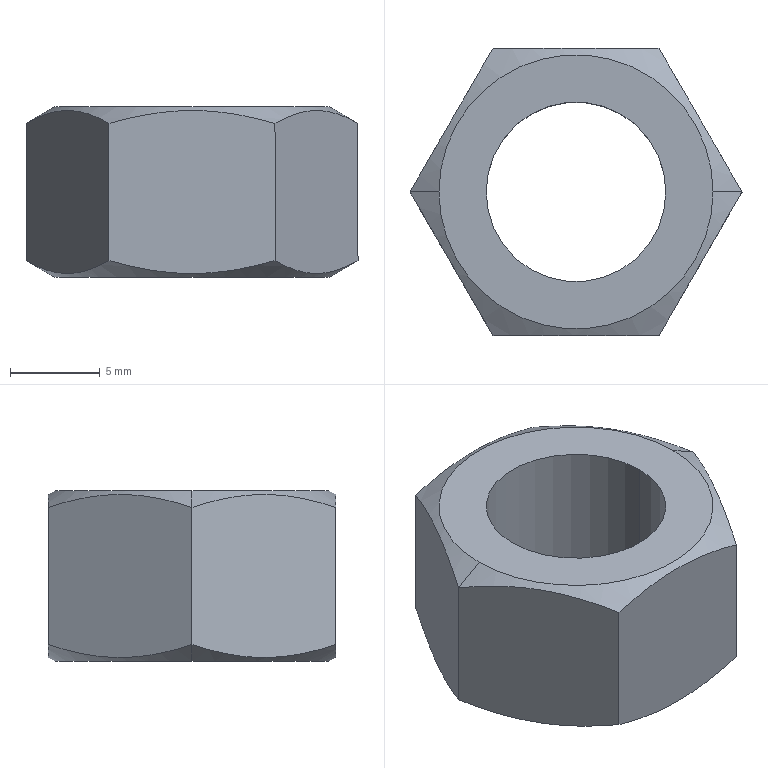Component | SolidWorks | hexagon nuts grade c gb-1 | 1 solid | 14 faces | box 18.48 x 16 x 9.5 mm | volume 1338 mm3 | plane 8 | cone 4 | cylinder 2 | commonest cylinder face diameters 10 x2
STEP:
#1=COLOUR_RGB('',0.7922,0.8196,0.9333);
#2=FILL_AREA_STYLE_COLOUR('',#1);
#3=FILL_AREA_STYLE('',(#2));
#4=SURFACE_STYLE_FILL_AREA(#3);
#5=SURFACE_SIDE_STYLE('',(#4));
#6=SURFACE_STYLE_USAGE(.BOTH.,#5);
#7=PRESENTATION_STYLE_ASSIGNMENT((#6));
#8=CARTESIAN_POINT('',(2.439,-3.29,-4.35));
#9=VERTEX_POINT('',#8);
#10=CARTESIAN_POINT('',(3.039,-3.29,-4.35));
#11=VERTEX_POINT('',#10);
#12=CARTESIAN_POINT('',(2.739,-3.29,-4.35));
#13=DIRECTION('',(0.,0.,-1.));
#14=DIRECTION('',(-1.,0.,0.));
#15=AXIS2_PLACEMENT_3D('',#12,#13,#14);
#16=CIRCLE('',#15,0.3002);
#17=EDGE_CURVE('',#9,#11,#16,.T.);
#18=ORIENTED_EDGE('',*,*,#17,.T.);
#19=CARTESIAN_POINT('',(3.103,-3.29,-4.387));
#20=VERTEX_POINT('',#19);
#21=CARTESIAN_POINT('',(3.039,-3.29,-4.35));
#22=DIRECTION('',(0.866,0.,-0.5));
#23=VECTOR('',#22,39.37);
#24=LINE('',#21,#23);
#25=EDGE_CURVE('',#11,#20,#24,.T.);
#26=ORIENTED_EDGE('',*,*,#25,.T.);
#27=CARTESIAN_POINT('',(2.921,-2.975,-4.387));
#28=VERTEX_POINT('',#27);
#29=CARTESIAN_POINT('',(3.103,-3.29,-4.387));
#30=CARTESIAN_POINT('',(3.088,-3.264,-4.378));
#31=CARTESIAN_POINT('',(3.073,-3.238,-4.371));
#32=CARTESIAN_POINT('',(3.043,-3.186,-4.362));
#33=CARTESIAN_POINT('',(3.027,-3.159,-4.359));
#34=CARTESIAN_POINT('',(3.004,-3.119,-4.359));
#35=CARTESIAN_POINT('',(2.996,-3.106,-4.36));
#36=CARTESIAN_POINT('',(2.981,-3.079,-4.362));
#37=CARTESIAN_POINT('',(2.973,-3.066,-4.364));
#38=CARTESIAN_POINT('',(2.951,-3.027,-4.371));
#39=CARTESIAN_POINT('',(2.936,-3.001,-4.378));
#40=CARTESIAN_POINT('',(2.921,-2.975,-4.387));
#41=B_SPLINE_CURVE_WITH_KNOTS('',3,(#29,#30,#31,#32,#33,#34,#35,#36,#37,#38,#39,#40),.UNSPECIFIED.,.F.,.F.,(4,2,2,2,2,4),(0.00000024,0.002333,0.004665,0.005831,0.006997,0.00933),.UNSPECIFIED.);
#42=EDGE_CURVE('',#20,#28,#41,.T.);
#43=ORIENTED_EDGE('',*,*,#42,.T.);
#44=CARTESIAN_POINT('',(2.557,-2.975,-4.387));
#45=VERTEX_POINT('',#44);
#46=CARTESIAN_POINT('',(2.921,-2.975,-4.387));
#47=CARTESIAN_POINT('',(2.891,-2.975,-4.379));
#48=CARTESIAN_POINT('',(2.862,-2.975,-4.371));
#49=CARTESIAN_POINT('',(2.801,-2.975,-4.362));
#50=CARTESIAN_POINT('',(2.77,-2.975,-4.359));
#51=CARTESIAN_POINT('',(2.708,-2.975,-4.359));
#52=CARTESIAN_POINT('',(2.678,-2.975,-4.362));
#53=CARTESIAN_POINT('',(2.617,-2.975,-4.371));
#54=CARTESIAN_POINT('',(2.587,-2.975,-4.379));
#55=CARTESIAN_POINT('',(2.557,-2.975,-4.387));
#56=B_SPLINE_CURVE_WITH_KNOTS('',3,(#46,#47,#48,#49,#50,#51,#52,#53,#54,#55),.UNSPECIFIED.,.F.,.F.,(4,2,2,2,4),(0.003422,0.005753,0.008084,0.01041,0.01275),.UNSPECIFIED.);
#57=EDGE_CURVE('',#28,#45,#56,.T.);
#58=ORIENTED_EDGE('',*,*,#57,.T.);
#59=CARTESIAN_POINT('',(2.375,-3.29,-4.387));
#60=VERTEX_POINT('',#59);
#61=CARTESIAN_POINT('',(2.557,-2.975,-4.387));
#62=CARTESIAN_POINT('',(2.542,-3.001,-4.378));
#63=CARTESIAN_POINT('',(2.527,-3.026,-4.371));
#64=CARTESIAN_POINT('',(2.497,-3.079,-4.362));
#65=CARTESIAN_POINT('',(2.482,-3.105,-4.359));
#66=CARTESIAN_POINT('',(2.459,-3.145,-4.359));
#67=CARTESIAN_POINT('',(2.451,-3.159,-4.36));
#68=CARTESIAN_POINT('',(2.436,-3.185,-4.362));
#69=CARTESIAN_POINT('',(2.428,-3.199,-4.364));
#70=CARTESIAN_POINT('',(2.405,-3.238,-4.371));
#71=CARTESIAN_POINT('',(2.39,-3.264,-4.378));
#72=CARTESIAN_POINT('',(2.375,-3.29,-4.387));
#73=B_SPLINE_CURVE_WITH_KNOTS('',3,(#61,#62,#63,#64,#65,#66,#67,#68,#69,#70,#71,#72),.UNSPECIFIED.,.F.,.F.,(4,2,2,2,2,4),(0.00000024,0.002333,0.004665,0.005831,0.006997,0.00933),.UNSPECIFIED.);
#74=EDGE_CURVE('',#45,#60,#73,.T.);
#75=ORIENTED_EDGE('',*,*,#74,.T.);
#76=CARTESIAN_POINT('',(2.439,-3.29,-4.35));
#77=DIRECTION('',(-0.866,0.,-0.5));
#78=VECTOR('',#77,39.37);
#79=LINE('',#76,#78);
#80=EDGE_CURVE('',#9,#60,#79,.T.);
#81=ORIENTED_EDGE('',*,*,#80,.F.);
#82=EDGE_LOOP('',(#18,#26,#43,#58,#75,#81));
#83=FACE_OUTER_BOUND('',#82,.T.);
#84=CARTESIAN_POINT('',(2.739,-3.29,-4.35));
#85=DIRECTION('',(0.,0.,-1.));
#86=DIRECTION('',(-1.,0.,0.));
#87=AXIS2_PLACEMENT_3D('',#84,#85,#86);
#88=CONICAL_SURFACE('',#87,0.3002,1.047);
#89=ADVANCED_FACE('',(#83),#88,.T.);
#90=CARTESIAN_POINT('',(2.439,-3.29,-4.724));
#91=VERTEX_POINT('',#90);
#92=CARTESIAN_POINT('',(3.039,-3.29,-4.724));
#93=VERTEX_POINT('',#92);
#94=CARTESIAN_POINT('',(2.739,-3.29,-4.724));
#95=DIRECTION('',(0.,0.,-1.));
#96=DIRECTION('',(-1.,0.,0.));
#97=AXIS2_PLACEMENT_3D('',#94,#95,#96);
#98=CIRCLE('',#97,0.3002);
#99=EDGE_CURVE('',#91,#93,#98,.T.);
#100=ORIENTED_EDGE('',*,*,#99,.F.);
#101=CARTESIAN_POINT('',(2.375,-3.29,-4.688));
#102=VERTEX_POINT('',#101);
#103=CARTESIAN_POINT('',(2.375,-3.29,-4.688));
#104=DIRECTION('',(-0.866,0.,0.5));
#105=VECTOR('',#104,39.37);
#106=LINE('',#103,#105);
#107=EDGE_CURVE('',#91,#102,#106,.T.);
#108=ORIENTED_EDGE('',*,*,#107,.T.);
#109=CARTESIAN_POINT('',(2.557,-2.975,-4.688));
#110=VERTEX_POINT('',#109);
#111=CARTESIAN_POINT('',(2.375,-3.29,-4.688));
#112=CARTESIAN_POINT('',(2.39,-3.264,-4.696));
#113=CARTESIAN_POINT('',(2.405,-3.238,-4.703));
#114=CARTESIAN_POINT('',(2.435,-3.186,-4.713));
#115=CARTESIAN_POINT('',(2.451,-3.159,-4.716));
#116=CARTESIAN_POINT('',(2.474,-3.119,-4.716));
#117=CARTESIAN_POINT('',(2.482,-3.106,-4.715));
#118=CARTESIAN_POINT('',(2.497,-3.079,-4.713));
#119=CARTESIAN_POINT('',(2.505,-3.066,-4.711));
#120=CARTESIAN_POINT('',(2.527,-3.027,-4.703));
#121=CARTESIAN_POINT('',(2.542,-3.001,-4.696));
#122=CARTESIAN_POINT('',(2.557,-2.975,-4.688));
#123=B_SPLINE_CURVE_WITH_KNOTS('',3,(#111,#112,#113,#114,#115,#116,#117,#118,#119,#120,#121,#122),.UNSPECIFIED.,.F.,.F.,(4,2,2,2,2,4),(0.00000024,0.002333,0.004665,0.005831,0.006997,0.00933),.UNSPECIFIED.);
#124=EDGE_CURVE('',#102,#110,#123,.T.);
#125=ORIENTED_EDGE('',*,*,#124,.T.);
#126=CARTESIAN_POINT('',(2.921,-2.975,-4.688));
#127=VERTEX_POINT('',#126);
#128=CARTESIAN_POINT('',(2.557,-2.975,-4.688));
#129=CARTESIAN_POINT('',(2.587,-2.975,-4.696));
#130=CARTESIAN_POINT('',(2.617,-2.975,-4.703));
#131=CARTESIAN_POINT('',(2.678,-2.975,-4.713));
#132=CARTESIAN_POINT('',(2.708,-2.975,-4.716));
#133=CARTESIAN_POINT('',(2.77,-2.975,-4.716));
#134=CARTESIAN_POINT('',(2.801,-2.975,-4.713));
#135=CARTESIAN_POINT('',(2.862,-2.975,-4.703));
#136=CARTESIAN_POINT('',(2.891,-2.975,-4.696));
#137=CARTESIAN_POINT('',(2.921,-2.975,-4.688));
#138=B_SPLINE_CURVE_WITH_KNOTS('',3,(#128,#129,#130,#131,#132,#133,#134,#135,#136,#137),.UNSPECIFIED.,.F.,.F.,(4,2,2,2,4),(0.008207,0.01054,0.01288,0.01522,0.01755),.UNSPECIFIED.);
#139=EDGE_CURVE('',#110,#127,#138,.T.);
#140=ORIENTED_EDGE('',*,*,#139,.T.);
#141=CARTESIAN_POINT('',(3.103,-3.29,-4.688));
#142=VERTEX_POINT('',#141);
#143=CARTESIAN_POINT('',(2.921,-2.975,-4.688));
#144=CARTESIAN_POINT('',(2.936,-3.001,-4.696));
#145=CARTESIAN_POINT('',(2.951,-3.026,-4.703));
#146=CARTESIAN_POINT('',(2.981,-3.079,-4.713));
#147=CARTESIAN_POINT('',(2.996,-3.105,-4.716));
#148=CARTESIAN_POINT('',(3.019,-3.145,-4.716));
#149=CARTESIAN_POINT('',(3.027,-3.159,-4.715));
#150=CARTESIAN_POINT('',(3.042,-3.185,-4.713));
#151=CARTESIAN_POINT('',(3.05,-3.199,-4.711));
#152=CARTESIAN_POINT('',(3.073,-3.238,-4.703));
#153=CARTESIAN_POINT('',(3.088,-3.264,-4.696));
#154=CARTESIAN_POINT('',(3.103,-3.29,-4.688));
#155=B_SPLINE_CURVE_WITH_KNOTS('',3,(#143,#144,#145,#146,#147,#148,#149,#150,#151,#152,#153,#154),.UNSPECIFIED.,.F.,.F.,(4,2,2,2,2,4),(0.00000024,0.002333,0.004665,0.005831,0.006997,0.00933),.UNSPECIFIED.);
#156=EDGE_CURVE('',#127,#142,#155,.T.);
#157=ORIENTED_EDGE('',*,*,#156,.T.);
#158=CARTESIAN_POINT('',(3.103,-3.29,-4.688));
#159=DIRECTION('',(0.866,0.,0.5));
#160=VECTOR('',#159,39.37);
#161=LINE('',#158,#160);
#162=EDGE_CURVE('',#93,#142,#161,.T.);
#163=ORIENTED_EDGE('',*,*,#162,.F.);
#164=EDGE_LOOP('',(#100,#108,#125,#140,#157,#163));
#165=FACE_OUTER_BOUND('',#164,.T.);
#166=CARTESIAN_POINT('',(2.739,-3.29,-4.688));
#167=DIRECTION('',(0.,0.,1.));
#168=DIRECTION('',(1.,0.,0.));
#169=AXIS2_PLACEMENT_3D('',#166,#167,#168);
#170=CONICAL_SURFACE('',#169,0.3637,1.047);
#171=ADVANCED_FACE('',(#165),#170,.T.);
#172=CARTESIAN_POINT('',(2.542,-3.29,-4.724));
#173=VERTEX_POINT('',#172);
#174=CARTESIAN_POINT('',(2.936,-3.29,-4.724));
#175=VERTEX_POINT('',#174);
#176=CARTESIAN_POINT('',(2.739,-3.29,-4.724));
#177=DIRECTION('',(0.,0.,1.));
#178=DIRECTION('',(1.,0.,0.));
#179=AXIS2_PLACEMENT_3D('',#176,#177,#178);
#180=CIRCLE('',#179,0.1969);
#181=EDGE_CURVE('',#173,#175,#180,.T.);
#182=ORIENTED_EDGE('',*,*,#181,.F.);
#183=CARTESIAN_POINT('',(2.542,-3.29,-4.35));
#184=VERTEX_POINT('',#183);
#185=CARTESIAN_POINT('',(2.542,-3.29,-4.724));
#186=DIRECTION('',(0.,0.,1.));
#187=VECTOR('',#186,39.37);
#188=LINE('',#185,#187);
#189=EDGE_CURVE('',#173,#184,#188,.T.);
#190=ORIENTED_EDGE('',*,*,#189,.T.);
#191=CARTESIAN_POINT('',(2.936,-3.29,-4.35));
#192=VERTEX_POINT('',#191);
#193=CARTESIAN_POINT('',(2.739,-3.29,-4.35));
#194=DIRECTION('',(0.,0.,1.));
#195=DIRECTION('',(1.,0.,0.));
#196=AXIS2_PLACEMENT_3D('',#193,#194,#195);
#197=CIRCLE('',#196,0.1969);
#198=EDGE_CURVE('',#184,#192,#197,.T.);
#199=ORIENTED_EDGE('',*,*,#198,.T.);
#200=CARTESIAN_POINT('',(2.936,-3.29,-4.724));
#201=DIRECTION('',(0.,0.,1.));
#202=VECTOR('',#201,39.37);
#203=LINE('',#200,#202);
#204=EDGE_CURVE('',#175,#192,#203,.T.);
#205=ORIENTED_EDGE('',*,*,#204,.F.);
#206=EDGE_LOOP('',(#182,#190,#199,#205));
#207=FACE_OUTER_BOUND('',#206,.T.);
#208=CARTESIAN_POINT('',(2.739,-3.29,-4.724));
#209=DIRECTION('',(0.,0.,1.));
#210=DIRECTION('',(1.,0.,0.));
#211=AXIS2_PLACEMENT_3D('',#208,#209,#210);
#212=CYLINDRICAL_SURFACE('',#211,0.1969);
#213=ADVANCED_FACE('',(#207),#212,.F.);
#214=CARTESIAN_POINT('',(2.557,-3.605,-4.387));
#215=VERTEX_POINT('',#214);
#216=CARTESIAN_POINT('',(2.921,-3.605,-4.387));
#217=VERTEX_POINT('',#216);
#218=CARTESIAN_POINT('',(2.557,-3.605,-4.387));
#219=CARTESIAN_POINT('',(2.587,-3.605,-4.379));
#220=CARTESIAN_POINT('',(2.617,-3.605,-4.371));
#221=CARTESIAN_POINT('',(2.678,-3.605,-4.362));
#222=CARTESIAN_POINT('',(2.708,-3.605,-4.359));
#223=CARTESIAN_POINT('',(2.77,-3.605,-4.359));
#224=CARTESIAN_POINT('',(2.801,-3.605,-4.362));
#225=CARTESIAN_POINT('',(2.862,-3.605,-4.371));
#226=CARTESIAN_POINT('',(2.891,-3.605,-4.379));
#227=CARTESIAN_POINT('',(2.921,-3.605,-4.387));
#228=B_SPLINE_CURVE_WITH_KNOTS('',3,(#218,#219,#220,#221,#222,#223,#224,#225,#226,#227),.UNSPECIFIED.,.F.,.F.,(4,2,2,2,4),(0.008207,0.01054,0.01288,0.01522,0.01755),.UNSPECIFIED.);
#229=EDGE_CURVE('',#215,#217,#228,.T.);
#230=ORIENTED_EDGE('',*,*,#229,.F.);
#231=CARTESIAN_POINT('',(2.557,-3.605,-4.688));
#232=VERTEX_POINT('',#231);
#233=CARTESIAN_POINT('',(2.557,-3.605,-4.724));
#234=DIRECTION('',(0.,0.,1.));
#235=VECTOR('',#234,39.37);
#236=LINE('',#233,#235);
#237=EDGE_CURVE('',#232,#215,#236,.T.);
#238=ORIENTED_EDGE('',*,*,#237,.F.);
#239=CARTESIAN_POINT('',(2.921,-3.605,-4.688));
#240=VERTEX_POINT('',#239);
#241=CARTESIAN_POINT('',(2.921,-3.605,-4.688));
#242=CARTESIAN_POINT('',(2.891,-3.605,-4.696));
#243=CARTESIAN_POINT('',(2.862,-3.605,-4.703));
#244=CARTESIAN_POINT('',(2.801,-3.605,-4.713));
#245=CARTESIAN_POINT('',(2.77,-3.605,-4.716));
#246=CARTESIAN_POINT('',(2.708,-3.605,-4.716));
#247=CARTESIAN_POINT('',(2.678,-3.605,-4.713));
#248=CARTESIAN_POINT('',(2.617,-3.605,-4.703));
#249=CARTESIAN_POINT('',(2.587,-3.605,-4.696));
#250=CARTESIAN_POINT('',(2.557,-3.605,-4.688));
#251=B_SPLINE_CURVE_WITH_KNOTS('',3,(#241,#242,#243,#244,#245,#246,#247,#248,#249,#250),.UNSPECIFIED.,.F.,.F.,(4,2,2,2,4),(0.003422,0.005753,0.008084,0.01041,0.01275),.UNSPECIFIED.);
#252=EDGE_CURVE('',#240,#232,#251,.T.);
#253=ORIENTED_EDGE('',*,*,#252,.F.);
#254=CARTESIAN_POINT('',(2.921,-3.605,-4.724));
#255=DIRECTION('',(0.,0.,1.));
#256=VECTOR('',#255,39.37);
#257=LINE('',#254,#256);
#258=EDGE_CURVE('',#240,#217,#257,.T.);
#259=ORIENTED_EDGE('',*,*,#258,.T.);
#260=EDGE_LOOP('',(#230,#238,#253,#259));
#261=FACE_OUTER_BOUND('',#260,.T.);
#262=CARTESIAN_POINT('',(2.557,-3.605,-4.724));
#263=DIRECTION('',(0.,-1.,0.));
#264=DIRECTION('',(0.,0.,-1.));
#265=AXIS2_PLACEMENT_3D('',#262,#263,#264);
#266=PLANE('',#265);
#267=ADVANCED_FACE('',(#261),#266,.T.);
#268=CARTESIAN_POINT('',(2.375,-3.29,-4.387));
#269=CARTESIAN_POINT('',(2.39,-3.316,-4.378));
#270=CARTESIAN_POINT('',(2.405,-3.341,-4.371));
#271=CARTESIAN_POINT('',(2.435,-3.394,-4.362));
#272=CARTESIAN_POINT('',(2.451,-3.42,-4.359));
#273=CARTESIAN_POINT('',(2.474,-3.46,-4.359));
#274=CARTESIAN_POINT('',(2.482,-3.474,-4.36));
#275=CARTESIAN_POINT('',(2.497,-3.5,-4.362));
#276=CARTESIAN_POINT('',(2.505,-3.514,-4.364));
#277=CARTESIAN_POINT('',(2.527,-3.553,-4.371));
#278=CARTESIAN_POINT('',(2.542,-3.579,-4.378));
#279=CARTESIAN_POINT('',(2.557,-3.605,-4.387));
#280=B_SPLINE_CURVE_WITH_KNOTS('',3,(#268,#269,#270,#271,#272,#273,#274,#275,#276,#277,#278,#279),.UNSPECIFIED.,.F.,.F.,(4,2,2,2,2,4),(0.00000024,0.002333,0.004665,0.005831,0.006997,0.00933),.UNSPECIFIED.);
#281=EDGE_CURVE('',#60,#215,#280,.T.);
#282=ORIENTED_EDGE('',*,*,#281,.F.);
#283=CARTESIAN_POINT('',(2.375,-3.29,-4.724));
#284=DIRECTION('',(0.,0.,1.));
#285=VECTOR('',#284,39.37);
#286=LINE('',#283,#285);
#287=EDGE_CURVE('',#102,#60,#286,.T.);
#288=ORIENTED_EDGE('',*,*,#287,.F.);
#289=CARTESIAN_POINT('',(2.557,-3.605,-4.688));
#290=CARTESIAN_POINT('',(2.542,-3.579,-4.696));
#291=CARTESIAN_POINT('',(2.527,-3.553,-4.703));
#292=CARTESIAN_POINT('',(2.497,-3.501,-4.713));
#293=CARTESIAN_POINT('',(2.482,-3.474,-4.716));
#294=CARTESIAN_POINT('',(2.459,-3.434,-4.716));
#295=CARTESIAN_POINT('',(2.451,-3.421,-4.715));
#296=CARTESIAN_POINT('',(2.436,-3.394,-4.713));
#297=CARTESIAN_POINT('',(2.428,-3.381,-4.711));
#298=CARTESIAN_POINT('',(2.405,-3.342,-4.703));
#299=CARTESIAN_POINT('',(2.39,-3.316,-4.696));
#300=CARTESIAN_POINT('',(2.375,-3.29,-4.688));
#301=B_SPLINE_CURVE_WITH_KNOTS('',3,(#289,#290,#291,#292,#293,#294,#295,#296,#297,#298,#299,#300),.UNSPECIFIED.,.F.,.F.,(4,2,2,2,2,4),(0.00000024,0.002333,0.004665,0.005831,0.006997,0.00933),.UNSPECIFIED.);
#302=EDGE_CURVE('',#232,#102,#301,.T.);
#303=ORIENTED_EDGE('',*,*,#302,.F.);
#304=ORIENTED_EDGE('',*,*,#237,.T.);
#305=EDGE_LOOP('',(#282,#288,#303,#304));
#306=FACE_OUTER_BOUND('',#305,.T.);
#307=CARTESIAN_POINT('',(2.375,-3.29,-4.724));
#308=DIRECTION('',(-0.866,-0.5,0.));
#309=DIRECTION('',(0.5,-0.866,0.));
#310=AXIS2_PLACEMENT_3D('',#307,#308,#309);
#311=PLANE('',#310);
#312=ADVANCED_FACE('',(#306),#311,.T.);
#313=ORIENTED_EDGE('',*,*,#74,.F.);
#314=CARTESIAN_POINT('',(2.557,-2.975,-4.724));
#315=DIRECTION('',(0.,0.,1.));
#316=VECTOR('',#315,39.37);
#317=LINE('',#314,#316);
#318=EDGE_CURVE('',#110,#45,#317,.T.);
#319=ORIENTED_EDGE('',*,*,#318,.F.);
#320=ORIENTED_EDGE('',*,*,#124,.F.);
#321=ORIENTED_EDGE('',*,*,#287,.T.);
#322=EDGE_LOOP('',(#313,#319,#320,#321));
#323=FACE_OUTER_BOUND('',#322,.T.);
#324=CARTESIAN_POINT('',(2.557,-2.975,-4.724));
#325=DIRECTION('',(-0.866,0.5,0.));
#326=DIRECTION('',(-0.5,-0.866,0.));
#327=AXIS2_PLACEMENT_3D('',#324,#325,#326);
#328=PLANE('',#327);
#329=ADVANCED_FACE('',(#323),#328,.T.);
#330=ORIENTED_EDGE('',*,*,#57,.F.);
#331=CARTESIAN_POINT('',(2.921,-2.975,-4.724));
#332=DIRECTION('',(0.,0.,1.));
#333=VECTOR('',#332,39.37);
#334=LINE('',#331,#333);
#335=EDGE_CURVE('',#127,#28,#334,.T.);
#336=ORIENTED_EDGE('',*,*,#335,.F.);
#337=ORIENTED_EDGE('',*,*,#139,.F.);
#338=ORIENTED_EDGE('',*,*,#318,.T.);
#339=EDGE_LOOP('',(#330,#336,#337,#338));
#340=FACE_OUTER_BOUND('',#339,.T.);
#341=CARTESIAN_POINT('',(2.921,-2.975,-4.724));
#342=DIRECTION('',(0.,1.,0.));
#343=DIRECTION('',(0.,0.,1.));
#344=AXIS2_PLACEMENT_3D('',#341,#342,#343);
#345=PLANE('',#344);
#346=ADVANCED_FACE('',(#340),#345,.T.);
#347=ORIENTED_EDGE('',*,*,#42,.F.);
#348=CARTESIAN_POINT('',(3.103,-3.29,-4.724));
#349=DIRECTION('',(0.,0.,1.));
#350=VECTOR('',#349,39.37);
#351=LINE('',#348,#350);
#352=EDGE_CURVE('',#142,#20,#351,.T.);
#353=ORIENTED_EDGE('',*,*,#352,.F.);
#354=ORIENTED_EDGE('',*,*,#156,.F.);
#355=ORIENTED_EDGE('',*,*,#335,.T.);
#356=EDGE_LOOP('',(#347,#353,#354,#355));
#357=FACE_OUTER_BOUND('',#356,.T.);
#358=CARTESIAN_POINT('',(3.103,-3.29,-4.724));
#359=DIRECTION('',(0.866,0.5,0.));
#360=DIRECTION('',(-0.5,0.866,0.));
#361=AXIS2_PLACEMENT_3D('',#358,#359,#360);
#362=PLANE('',#361);
#363=ADVANCED_FACE('',(#357),#362,.T.);
#364=CARTESIAN_POINT('',(2.921,-3.605,-4.387));
#365=CARTESIAN_POINT('',(2.936,-3.579,-4.378));
#366=CARTESIAN_POINT('',(2.951,-3.553,-4.371));
#367=CARTESIAN_POINT('',(2.981,-3.501,-4.362));
#368=CARTESIAN_POINT('',(2.996,-3.474,-4.359));
#369=CARTESIAN_POINT('',(3.019,-3.434,-4.359));
#370=CARTESIAN_POINT('',(3.027,-3.421,-4.36));
#371=CARTESIAN_POINT('',(3.042,-3.394,-4.362));
#372=CARTESIAN_POINT('',(3.05,-3.381,-4.364));
#373=CARTESIAN_POINT('',(3.073,-3.342,-4.371));
#374=CARTESIAN_POINT('',(3.088,-3.316,-4.378));
#375=CARTESIAN_POINT('',(3.103,-3.29,-4.387));
#376=B_SPLINE_CURVE_WITH_KNOTS('',3,(#364,#365,#366,#367,#368,#369,#370,#371,#372,#373,#374,#375),.UNSPECIFIED.,.F.,.F.,(4,2,2,2,2,4),(0.00000024,0.002333,0.004665,0.005831,0.006997,0.00933),.UNSPECIFIED.);
#377=EDGE_CURVE('',#217,#20,#376,.T.);
#378=ORIENTED_EDGE('',*,*,#377,.F.);
#379=ORIENTED_EDGE('',*,*,#258,.F.);
#380=CARTESIAN_POINT('',(3.103,-3.29,-4.688));
#381=CARTESIAN_POINT('',(3.088,-3.316,-4.696));
#382=CARTESIAN_POINT('',(3.073,-3.341,-4.703));
#383=CARTESIAN_POINT('',(3.043,-3.394,-4.713));
#384=CARTESIAN_POINT('',(3.027,-3.42,-4.716));
#385=CARTESIAN_POINT('',(3.004,-3.46,-4.716));
#386=CARTESIAN_POINT('',(2.996,-3.474,-4.715));
#387=CARTESIAN_POINT('',(2.981,-3.5,-4.713));
#388=CARTESIAN_POINT('',(2.973,-3.514,-4.711));
#389=CARTESIAN_POINT('',(2.951,-3.553,-4.703));
#390=CARTESIAN_POINT('',(2.936,-3.579,-4.696));
#391=CARTESIAN_POINT('',(2.921,-3.605,-4.688));
#392=B_SPLINE_CURVE_WITH_KNOTS('',3,(#380,#381,#382,#383,#384,#385,#386,#387,#388,#389,#390,#391),.UNSPECIFIED.,.F.,.F.,(4,2,2,2,2,4),(0.00000024,0.002333,0.004665,0.005831,0.006997,0.00933),.UNSPECIFIED.);
#393=EDGE_CURVE('',#142,#240,#392,.T.);
#394=ORIENTED_EDGE('',*,*,#393,.F.);
#395=ORIENTED_EDGE('',*,*,#352,.T.);
#396=EDGE_LOOP('',(#378,#379,#394,#395));
#397=FACE_OUTER_BOUND('',#396,.T.);
#398=CARTESIAN_POINT('',(2.921,-3.605,-4.724));
#399=DIRECTION('',(0.866,-0.5,0.));
#400=DIRECTION('',(0.5,0.866,0.));
#401=AXIS2_PLACEMENT_3D('',#398,#399,#400);
#402=PLANE('',#401);
#403=ADVANCED_FACE('',(#397),#402,.T.);
#404=CARTESIAN_POINT('',(2.739,-3.29,-4.724));
#405=DIRECTION('',(0.,0.,-1.));
#406=DIRECTION('',(-1.,0.,0.));
#407=AXIS2_PLACEMENT_3D('',#404,#405,#406);
#408=CIRCLE('',#407,0.3002);
#409=EDGE_CURVE('',#93,#91,#408,.T.);
#410=ORIENTED_EDGE('',*,*,#409,.T.);
#411=ORIENTED_EDGE('',*,*,#99,.T.);
#412=EDGE_LOOP('',(#410,#411));
#413=FACE_OUTER_BOUND('',#412,.T.);
#414=CARTESIAN_POINT('',(2.739,-3.29,-4.724));
#415=DIRECTION('',(0.,0.,1.));
#416=DIRECTION('',(1.,0.,0.));
#417=AXIS2_PLACEMENT_3D('',#414,#415,#416);
#418=CIRCLE('',#417,0.1969);
#419=EDGE_CURVE('',#175,#173,#418,.T.);
#420=ORIENTED_EDGE('',*,*,#419,.T.);
#421=ORIENTED_EDGE('',*,*,#181,.T.);
#422=EDGE_LOOP('',(#420,#421));
#423=FACE_BOUND('',#422,.T.);
#424=CARTESIAN_POINT('',(2.921,-3.605,-4.724));
#425=DIRECTION('',(0.,0.,1.));
#426=DIRECTION('',(1.,0.,0.));
#427=AXIS2_PLACEMENT_3D('',#424,#425,#426);
#428=PLANE('',#427);
#429=ADVANCED_FACE('',(#413,#423),#428,.F.);
#430=ORIENTED_EDGE('',*,*,#17,.F.);
#431=CARTESIAN_POINT('',(2.739,-3.29,-4.35));
#432=DIRECTION('',(0.,0.,-1.));
#433=DIRECTION('',(-1.,0.,0.));
#434=AXIS2_PLACEMENT_3D('',#431,#432,#433);
#435=CIRCLE('',#434,0.3002);
#436=EDGE_CURVE('',#11,#9,#435,.T.);
#437=ORIENTED_EDGE('',*,*,#436,.F.);
#438=EDGE_LOOP('',(#430,#437));
#439=FACE_OUTER_BOUND('',#438,.T.);
#440=CARTESIAN_POINT('',(2.739,-3.29,-4.35));
#441=DIRECTION('',(0.,0.,1.));
#442=DIRECTION('',(1.,0.,0.));
#443=AXIS2_PLACEMENT_3D('',#440,#441,#442);
#444=CIRCLE('',#443,0.1969);
#445=EDGE_CURVE('',#192,#184,#444,.T.);
#446=ORIENTED_EDGE('',*,*,#445,.F.);
#447=ORIENTED_EDGE('',*,*,#198,.F.);
#448=EDGE_LOOP('',(#446,#447));
#449=FACE_BOUND('',#448,.T.);
#450=CARTESIAN_POINT('',(2.921,-3.605,-4.35));
#451=DIRECTION('',(0.,0.,1.));
#452=DIRECTION('',(1.,0.,0.));
#453=AXIS2_PLACEMENT_3D('',#450,#451,#452);
#454=PLANE('',#453);
#455=ADVANCED_FACE('',(#439,#449),#454,.T.);
#456=ORIENTED_EDGE('',*,*,#189,.F.);
#457=ORIENTED_EDGE('',*,*,#419,.F.);
#458=ORIENTED_EDGE('',*,*,#204,.T.);
#459=ORIENTED_EDGE('',*,*,#445,.T.);
#460=EDGE_LOOP('',(#456,#457,#458,#459));
#461=FACE_OUTER_BOUND('',#460,.T.);
#462=CARTESIAN_POINT('',(2.739,-3.29,-4.724));
#463=DIRECTION('',(0.,0.,1.));
#464=DIRECTION('',(1.,0.,0.));
#465=AXIS2_PLACEMENT_3D('',#462,#463,#464);
#466=CYLINDRICAL_SURFACE('',#465,0.1969);
#467=ADVANCED_FACE('',(#461),#466,.F.);
#468=ORIENTED_EDGE('',*,*,#107,.F.);
#469=ORIENTED_EDGE('',*,*,#409,.F.);
#470=ORIENTED_EDGE('',*,*,#162,.T.);
#471=ORIENTED_EDGE('',*,*,#393,.T.);
#472=ORIENTED_EDGE('',*,*,#252,.T.);
#473=ORIENTED_EDGE('',*,*,#302,.T.);
#474=EDGE_LOOP('',(#468,#469,#470,#471,#472,#473));
#475=FACE_OUTER_BOUND('',#474,.T.);
#476=CARTESIAN_POINT('',(2.739,-3.29,-4.688));
#477=DIRECTION('',(0.,0.,1.));
#478=DIRECTION('',(1.,0.,0.));
#479=AXIS2_PLACEMENT_3D('',#476,#477,#478);
#480=CONICAL_SURFACE('',#479,0.3637,1.047);
#481=ADVANCED_FACE('',(#475),#480,.T.);
#482=ORIENTED_EDGE('',*,*,#25,.F.);
#483=ORIENTED_EDGE('',*,*,#436,.T.);
#484=ORIENTED_EDGE('',*,*,#80,.T.);
#485=ORIENTED_EDGE('',*,*,#281,.T.);
#486=ORIENTED_EDGE('',*,*,#229,.T.);
#487=ORIENTED_EDGE('',*,*,#377,.T.);
#488=EDGE_LOOP('',(#482,#483,#484,#485,#486,#487));
#489=FACE_OUTER_BOUND('',#488,.T.);
#490=CARTESIAN_POINT('',(2.739,-3.29,-4.35));
#491=DIRECTION('',(0.,0.,-1.));
#492=DIRECTION('',(-1.,0.,0.));
#493=AXIS2_PLACEMENT_3D('',#490,#491,#492);
#494=CONICAL_SURFACE('',#493,0.3002,1.047);
#495=ADVANCED_FACE('',(#489),#494,.T.);
#496=CLOSED_SHELL('',(#89,#171,#213,#267,#312,#329,#346,#363,#403,#429,#455,#467,#481,#495));
#497=MANIFOLD_SOLID_BREP('',#496);
#498=STYLED_ITEM('',(#7),#497);
#499=PRESENTATION_LAYER_ASSIGNMENT('','',(#498));
#500=(LENGTH_UNIT()NAMED_UNIT(*)SI_UNIT($,.METRE.));
#501=LENGTH_MEASURE_WITH_UNIT(LENGTH_MEASURE(0.0254),#500);
#502=DIMENSIONAL_EXPONENTS(1.,0.,0.,0.,0.,0.,0.);
#503=(CONVERSION_BASED_UNIT('',#501)LENGTH_UNIT()NAMED_UNIT(#502));
#504=UNCERTAINTY_MEASURE_WITH_UNIT(LENGTH_MEASURE(0.00001),#503,'','');
#505=(NAMED_UNIT(*)PLANE_ANGLE_UNIT()SI_UNIT($,.RADIAN.));
#506=(NAMED_UNIT(*)SI_UNIT($,.STERADIAN.)SOLID_ANGLE_UNIT());
#507=(GEOMETRIC_REPRESENTATION_CONTEXT(3)GLOBAL_UNCERTAINTY_ASSIGNED_CONTEXT((#504))GLOBAL_UNIT_ASSIGNED_CONTEXT((#503,#505,#506))REPRESENTATION_CONTEXT('',''));
#508=MECHANICAL_DESIGN_GEOMETRIC_PRESENTATION_REPRESENTATION('',(#498),#507);
#509=CARTESIAN_POINT('',(0.,0.,0.));
#510=DIRECTION('',(0.,0.,1.));
#511=DIRECTION('',(1.,0.,0.));
#512=AXIS2_PLACEMENT_3D('',#509,#510,#511);
#513=(LENGTH_UNIT()NAMED_UNIT(*)SI_UNIT($,.METRE.));
#514=LENGTH_MEASURE_WITH_UNIT(LENGTH_MEASURE(0.0254),#513);
#515=DIMENSIONAL_EXPONENTS(1.,0.,0.,0.,0.,0.,0.);
#516=(CONVERSION_BASED_UNIT('',#514)LENGTH_UNIT()NAMED_UNIT(#515));
#517=UNCERTAINTY_MEASURE_WITH_UNIT(LENGTH_MEASURE(0.00001),#516,'','');
#518=(NAMED_UNIT(*)PLANE_ANGLE_UNIT()SI_UNIT($,.RADIAN.));
#519=(NAMED_UNIT(*)SI_UNIT($,.STERADIAN.)SOLID_ANGLE_UNIT());
#520=(GEOMETRIC_REPRESENTATION_CONTEXT(3)GLOBAL_UNCERTAINTY_ASSIGNED_CONTEXT((#517))GLOBAL_UNIT_ASSIGNED_CONTEXT((#516,#518,#519))REPRESENTATION_CONTEXT('',''));
#521=ADVANCED_BREP_SHAPE_REPRESENTATION('',(#497,#512),#520);